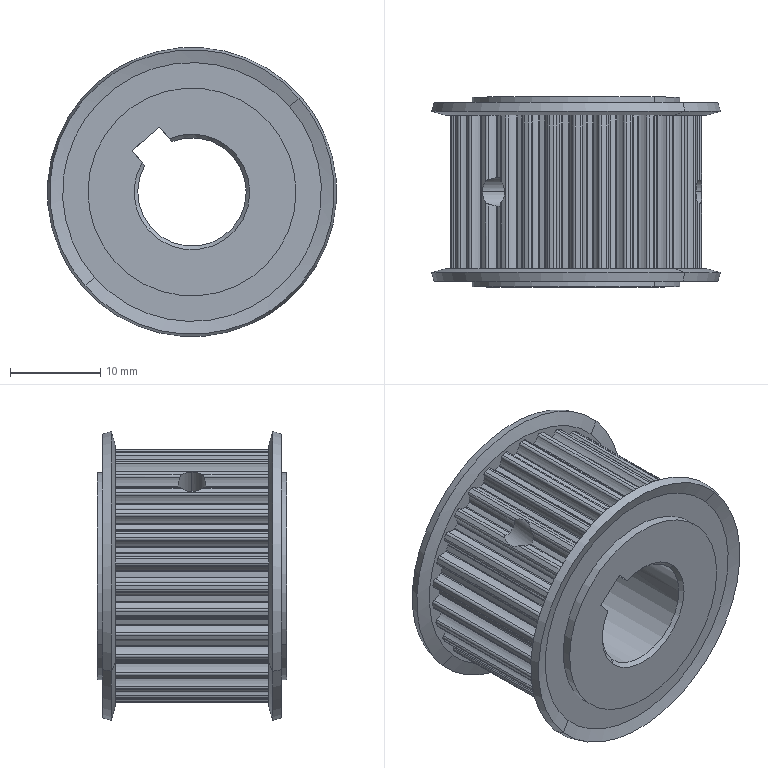Component | SolidWorks | EBF41-S3M150-30-A-N-d12.stp-1 | 1 solid | 320 faces | volume 9321 mm3 | cylinder 293 | cone 18 | plane 9 | commonest cylinder face diameters 0.56 x76 0.3 x73 3.95 x68 25.67 x32 27.89 x31 23 x4 3.242 x4 12 x3 | material 6061 Alloy